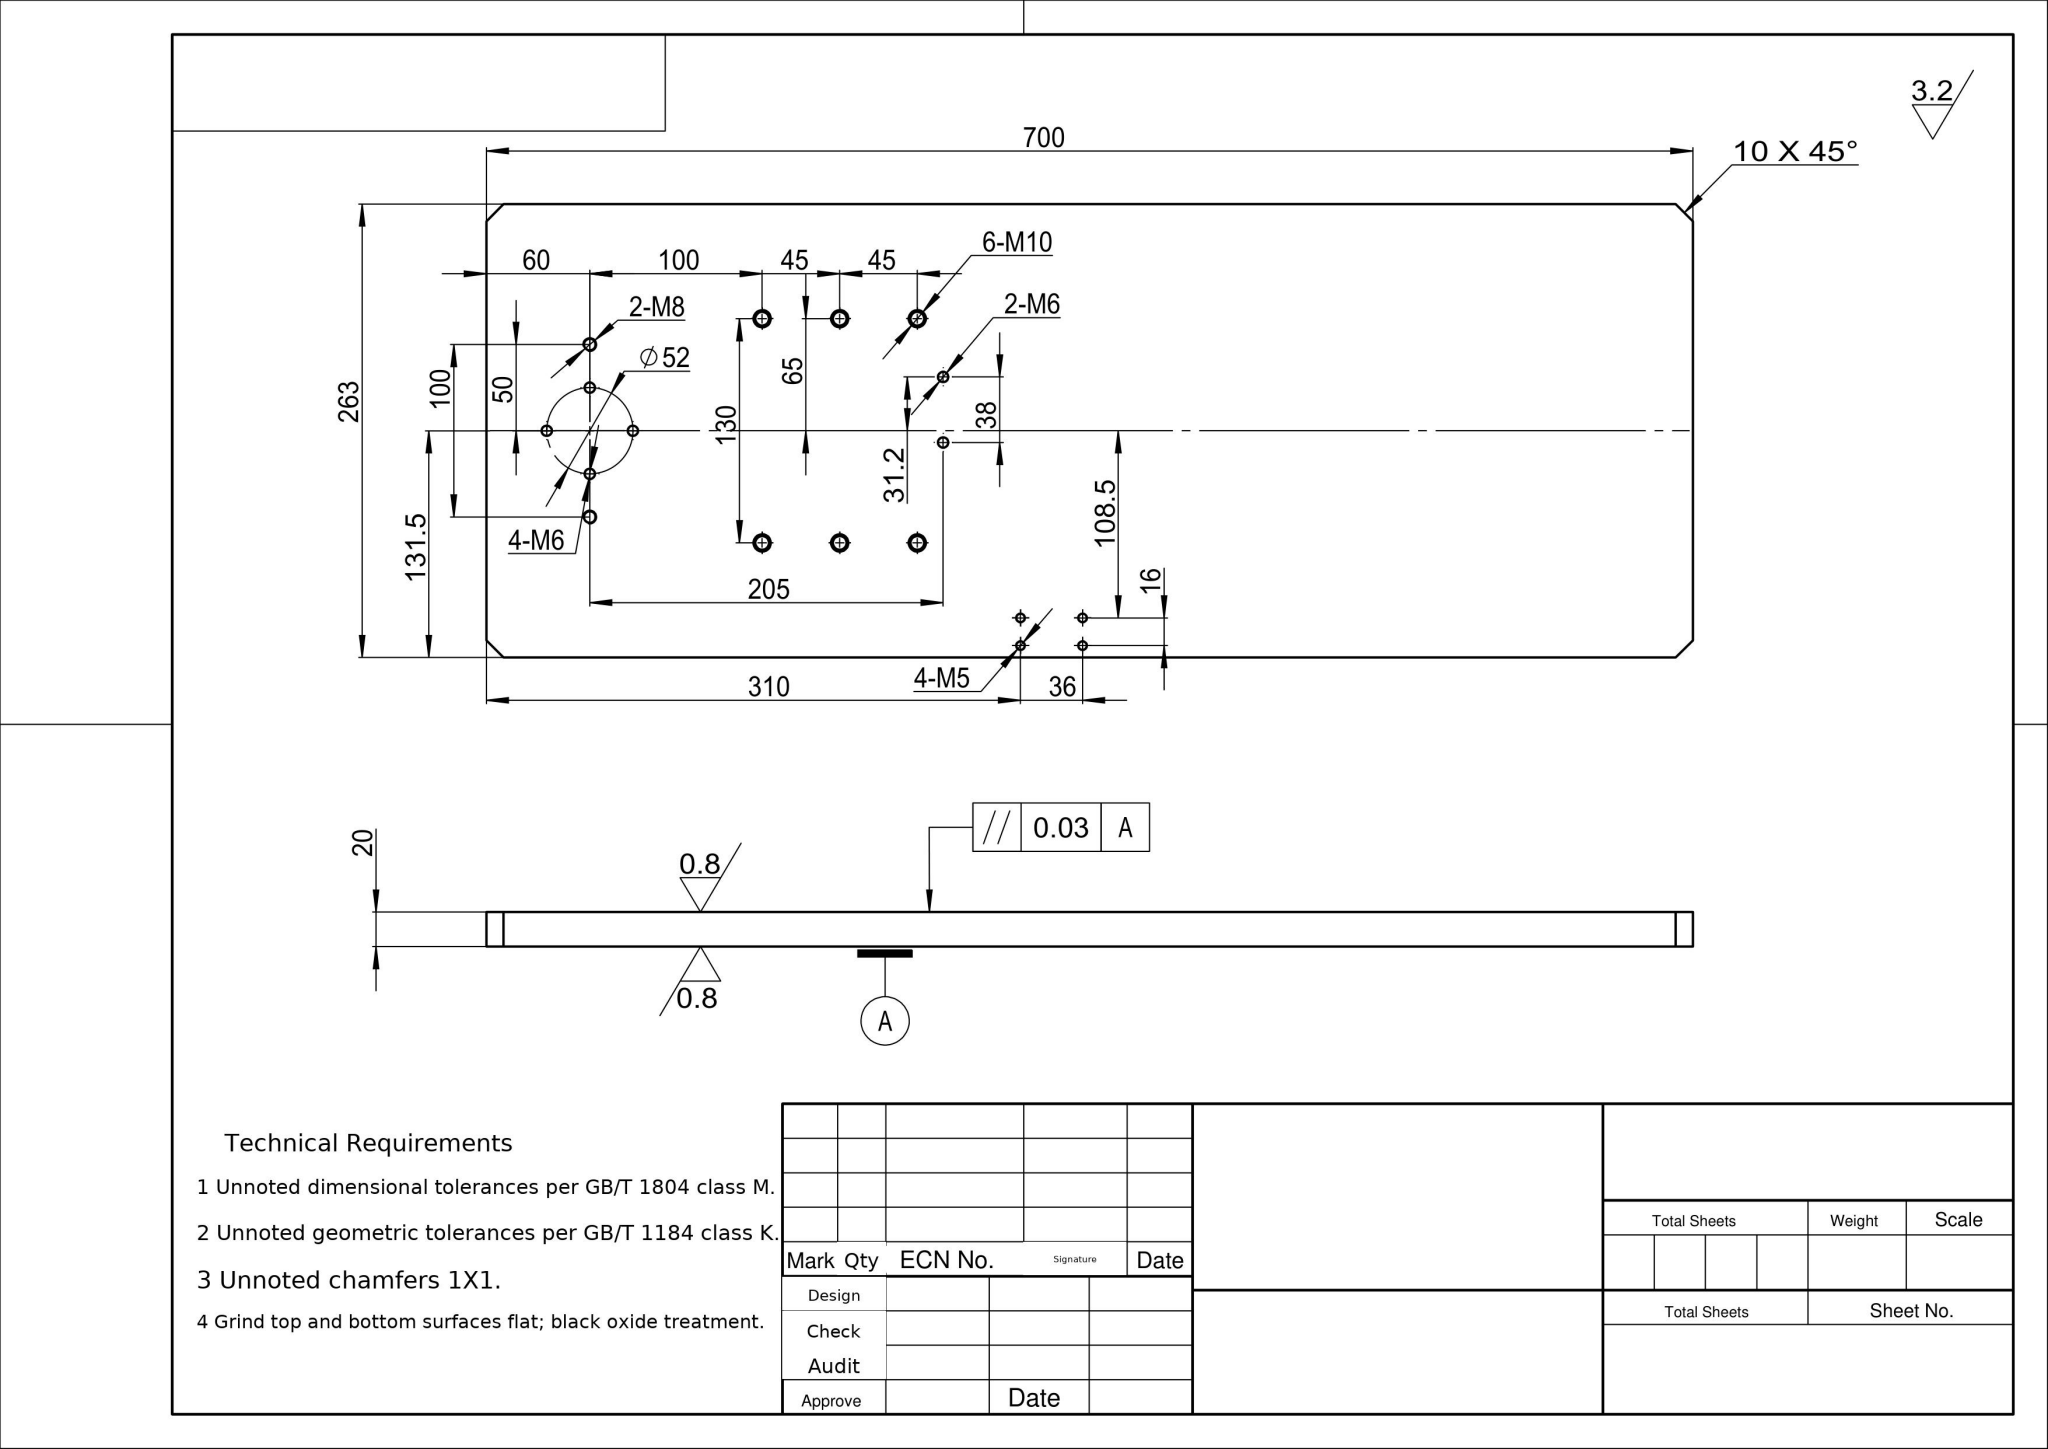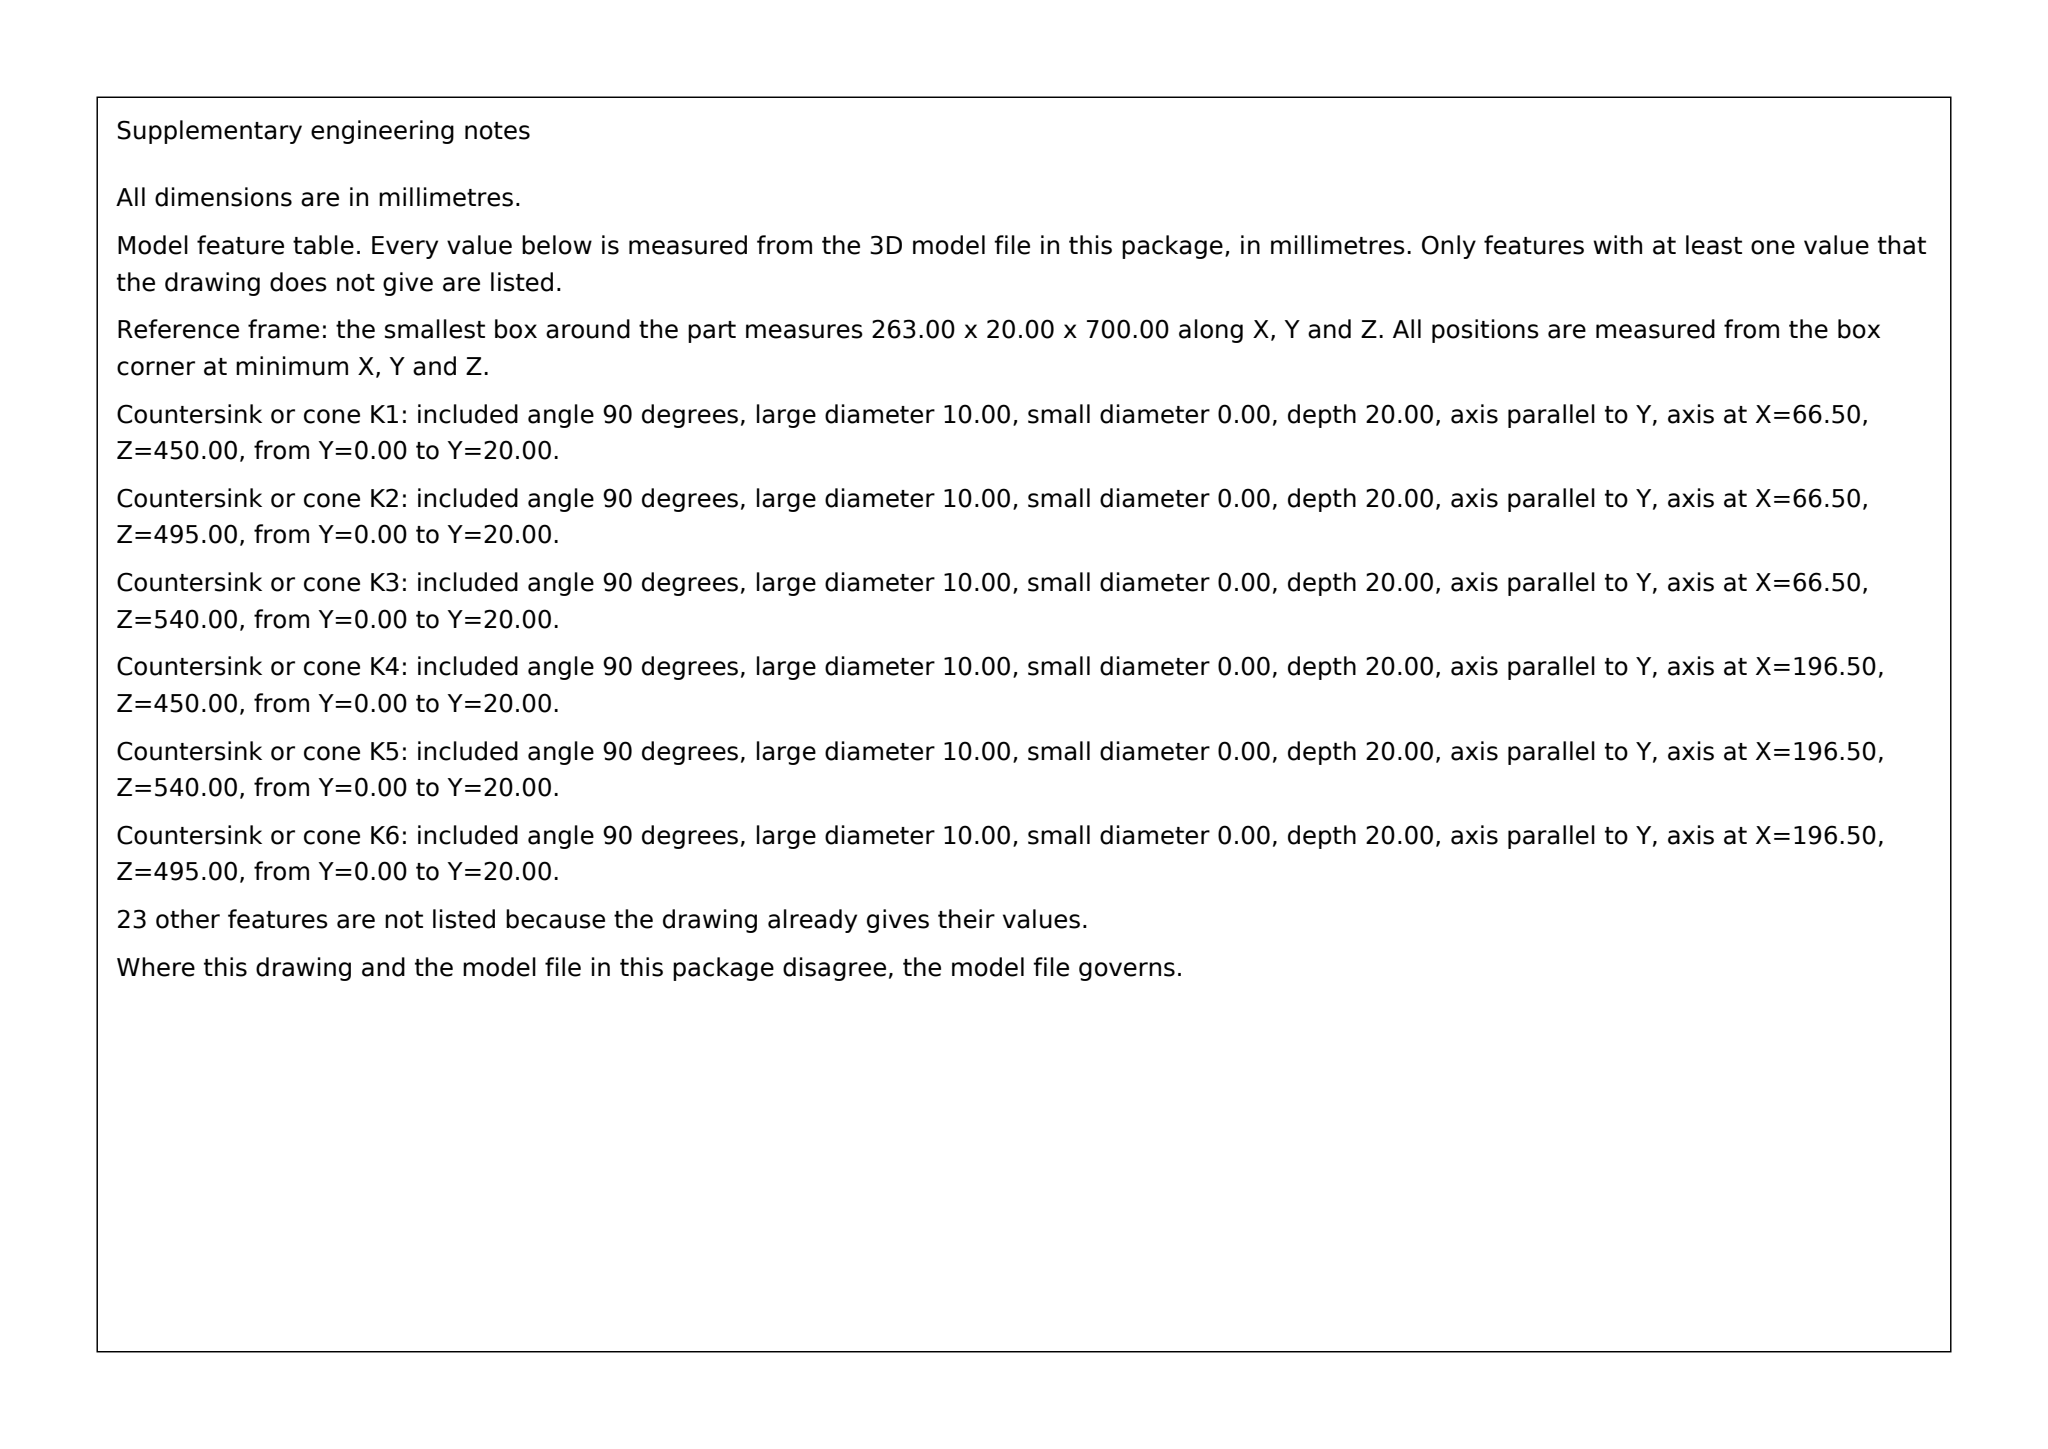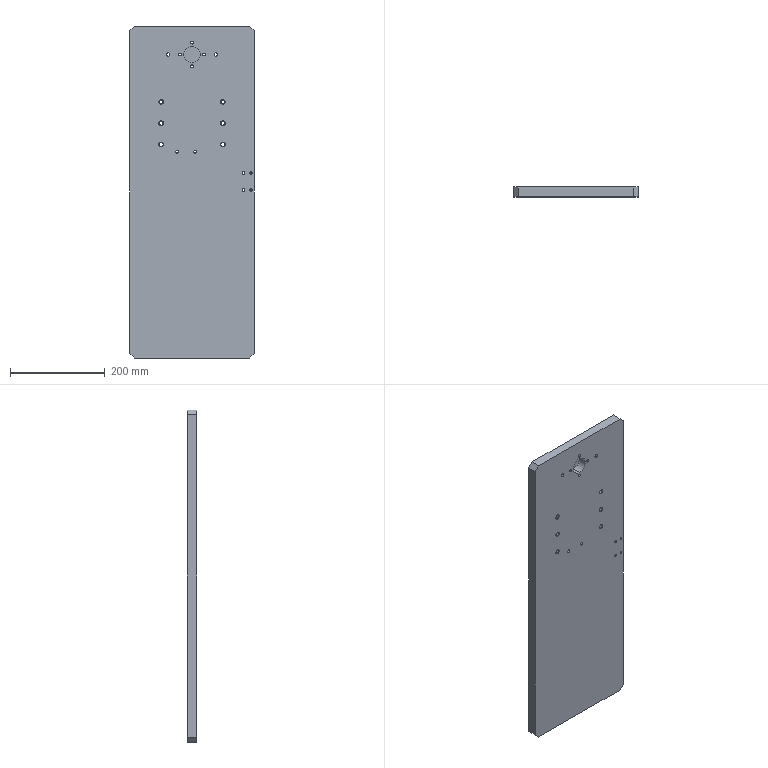Part | SolidWorks | mm | 1 solid | 73 faces | box 263 x 20 x 700 mm | volume 3648070 mm3 | cylinder 38 | cone 24 | plane 11 | commonest cylinder face diameters 6 x12 8 x12 5 x8 6.8 x4 35 x2
build123d program:
from build123d import *

# Parameters (mm, degrees)
SKETCH1_W           = 263
SKETCH1_H           = 20
BOSS_EXTRUDE1_DEPTH = 700
SKETCH2_R           = 17.5
SKETCH2_R_2         = 4
SKETCH2_R_3         = 3
CUT_EXTRUDE1_DEPTH  = 749.043
SKETCH3_R           = 2.5
CUT_EXTRUDE2_DEPTH  = 749.043
CHAMFER1_SIZE       = 10
SKETCH4_R           = 17.5
BOSS_EXTRUDE2_DEPTH = 2
CHAMFER2_SIZE       = 1
M8_TAPPED_HOLE1_D   = 6.8


with BuildPart() as part:
    # Sketch1 → Boss-Extrude1 (new body)
    with BuildSketch(Plane.XY):
        with Locations((131.5, -10)):
            Rectangle(SKETCH1_W, SKETCH1_H)
    extrude(amount=BOSS_EXTRUDE1_DEPTH)

    # Sketch2 → Cut-Extrude1 (cut, through all)
    with BuildSketch(Plane(origin=(0, 0, 0), x_dir=(1, 0, 0), z_dir=(0, 1, 0))):
        with Locations(Location((131.5, -640, 0), (0, 0, 270))):
            Circle(SKETCH2_R)
        with Locations(Location((66.5, -540, 0), (0, 0, 270))):
            Circle(SKETCH2_R_2)
        with Locations(Location((66.5, -495, 0), (0, 0, 270))):
            Circle(SKETCH2_R_2)
        with Locations(Location((66.5, -450, 0), (0, 0, 270))):
            Circle(SKETCH2_R_2)
        with Locations(Location((196.5, -450, 0), (0, 0, 270))):
            Circle(SKETCH2_R_2)
        with Locations(Location((196.5, -495, 0), (0, 0, 270))):
            Circle(SKETCH2_R_2)
        with Locations(Location((196.5, -540, 0), (0, 0, 270))):
            Circle(SKETCH2_R_2)
        with Locations(Location((100.3, -435, 0), (0, 0, 270))):
            Circle(SKETCH2_R_3)
        with Locations(Location((138.3, -435, 0), (0, 0, 270))):
            Circle(SKETCH2_R_3)
        with Locations(Location((131.5, -665, 0), (0, 0, 270))):
            Circle(SKETCH2_R_3)
        with Locations(Location((156.5, -640, 0), (0, 0, 270))):
            Circle(SKETCH2_R_3)
        with Locations(Location((131.5, -615, 0), (0, 0, 270))):
            Circle(SKETCH2_R_3)
        with Locations(Location((106.5, -640, 0), (0, 0, 270))):
            Circle(SKETCH2_R_3)
    extrude(amount=-CUT_EXTRUDE1_DEPTH, mode=Mode.SUBTRACT)

    # Sketch3 → Cut-Extrude2 (cut, through all)
    with BuildSketch(Plane(origin=(0, 0, 0), x_dir=(1, 0, 0), z_dir=(0, 1, 0))):
        with Locations(Location((256.05, -390.13, 0), (0, 0, 270))):
            Circle(SKETCH3_R)
        with Locations(Location((240.05, -390.13, 0), (0, 0, 270))):
            Circle(SKETCH3_R)
        with Locations(Location((256.05, -354.13, 0), (0, 0, 270))):
            Circle(SKETCH3_R)
        with Locations(Location((240.05, -354.13, 0), (0, 0, 270))):
            Circle(SKETCH3_R)
    extrude(amount=-CUT_EXTRUDE2_DEPTH, mode=Mode.SUBTRACT)

    # Chamfer1
    chamfer1_edges = [part.edges().sort_by_distance(p)[0] for p in [
        (263, -10, 700),
        (0, -10, 700),
        (263, -10, 0),
        (0, -10, 0),
    ]]
    chamfer(chamfer1_edges, length=CHAMFER1_SIZE)

    # Sketch4 → Boss-Extrude2 (add)
    with BuildSketch(Plane(origin=(0, 0, 0), x_dir=(1, 0, 0), z_dir=(0, 1, 0))):
        with Locations((131.5, -640)):
            Circle(SKETCH4_R)
    extrude(amount=-BOSS_EXTRUDE2_DEPTH)

    # Chamfer2
    chamfer2_edges = [part.edges().sort_by_distance(p)[0] for p in [
        (66.5, -20, 536),
        (66.5, 0, 536),
        (66.5, -20, 491),
        (66.5, 0, 491),
        (66.5, -20, 446),
        (66.5, 0, 446),
        (196.5, -20, 446),
        (196.5, 0, 446),
        (196.5, -20, 491),
        (196.5, 0, 491),
        (196.5, -20, 536),
        (196.5, 0, 536),
    ]]
    chamfer(chamfer2_edges, length=CHAMFER2_SIZE)

    # M8 Tapped Hole1 (through all)
    with Locations(Plane(origin=(0, 0, 0), x_dir=(-1, 0, 0), z_dir=(0, 1, 0))):
        with Locations((-81.5, 640), (-181.5, 640)):
            Hole(M8_TAPPED_HOLE1_D / 2)


solid = part.part